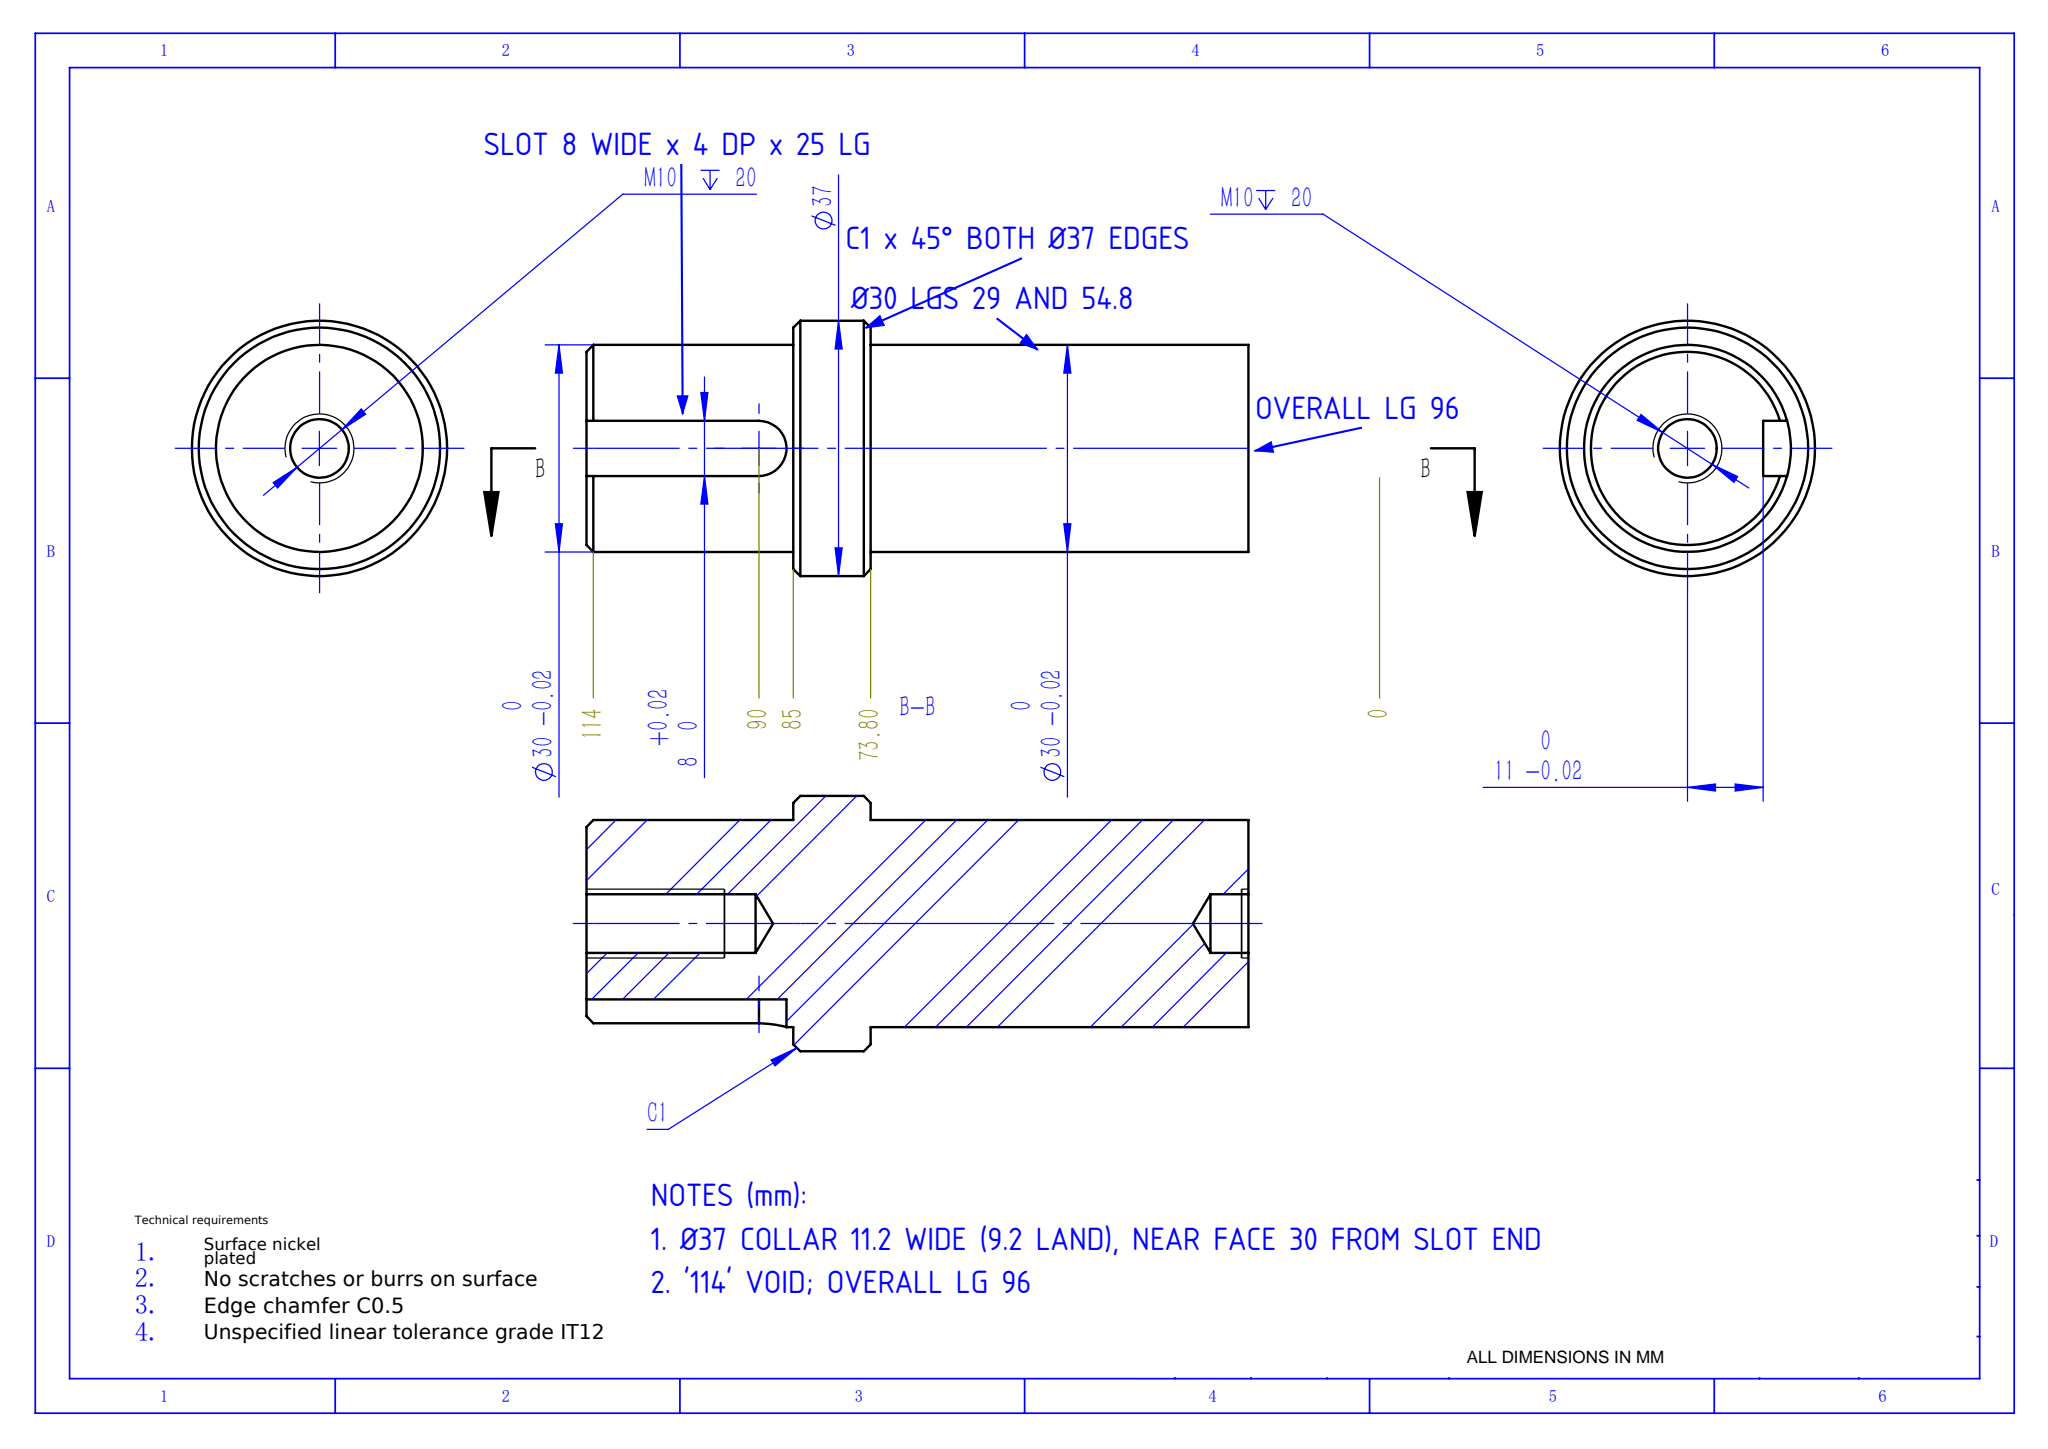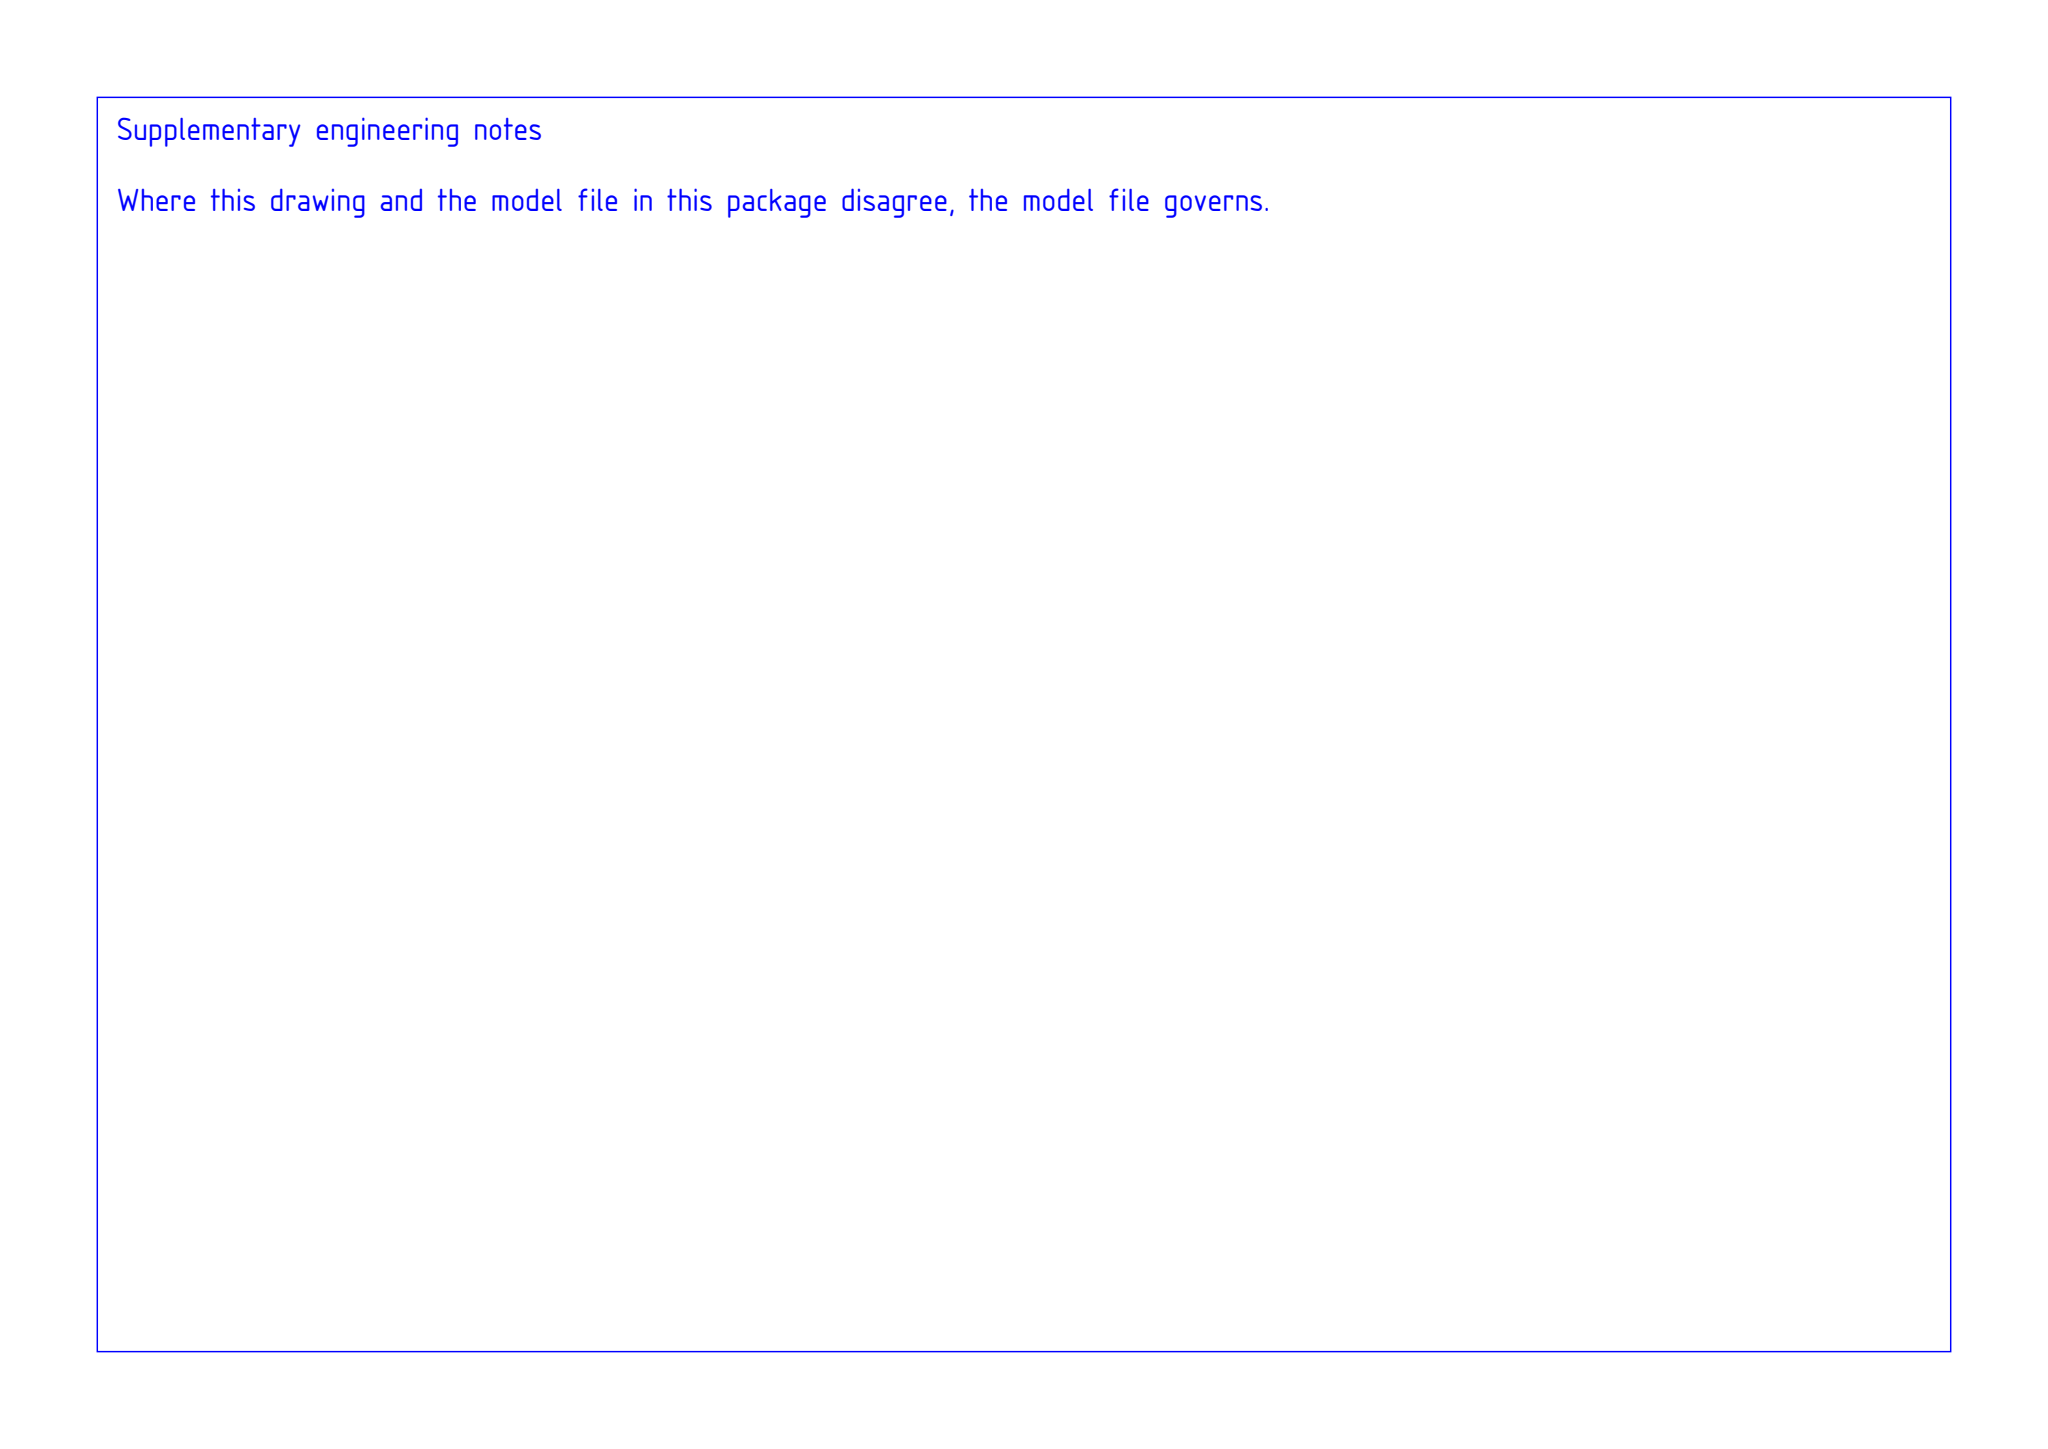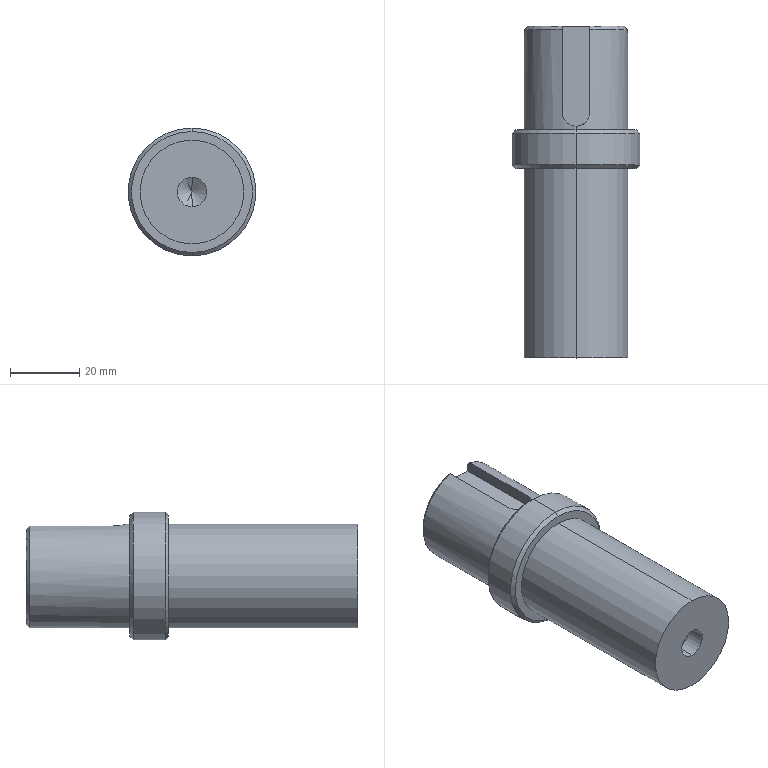Part | SolidWorks | mm | 1 solid | 28 faces | box 37 x 96 x 37 mm | volume 69168 mm3 | cylinder 11 | cone 10 | plane 7 | commonest cylinder face diameters 8.5 x4 30 x4 37 x2 8 x1
Drawing notes:
OVERALL LG 96 FROM LH END FACE; RH Ø30 SECTION 25.2 LG PAST FLANGE | from the solid: bbox_xyz y=96 overall; flange y=54.8..66.0 (Ø37 9.2 lg), Ø30 cyl y=66.0..96.0 => 30.0? RH face plane y=96.0, flange RH face y=66.0
Ø37 COLLAR 11.2 WIDE (9.2 LAND), NEAR FACE 30 FROM SLOT END | from the solid: Ø37 cyl len 9.2 between y-planes 54.8 and 66.0; end face y=96; 96-66=30
SLOT 8 WIDE x 4 DP x 25 LG FROM SLOT END FACE, R4 CLOSED END | from the solid: x-planes 14.5/22.5 = 8 wide; z-plane 29.5 vs Ø30 top 33.5 = 4 dp; Ø8 z-cyl at y=71 to end y=96 = 25, R4
Ø30 LGS: 29 SLOT END TO COLLAR, 54.8 COLLAR TO OPP END | from the solid: Ø30 cylinders len 29.0 (y 66-95) and 54.8 (y 0-54.8)
BOTH Ø37 COLLAR EDGES C1 x 45° (Ø37 TO Ø35) | from the solid: 90° cones ref dia 37 and 35 at collar faces = 1 mm chamfer
'114' VOID; OVERALL LG 96 | from the solid: bbox y = 96.0 overall
build123d program:
from build123d import *

# Parameters (mm, degrees)
SKETCH11_R             = 20
ROUND_STEEL_40_1_DEPTH = 115
M10_TAPPED_HOLE1_D     = 8.5
M10_TAPPED_HOLE1_DEPTH = 24.5
M10_TAPPED_HOLE1_TIP   = 2.554
CUT_EXTRUDE11_DEPTH    = 4
CHAMFER1_SIZE          = 1
M10_TAPPED_HOLE2_D     = 8.5
M10_TAPPED_HOLE2_DEPTH = 24.5
M10_TAPPED_HOLE2_TIP   = 2.554
SKETCH14_R             = 24.282
CUT_EXTRUDE1_DEPTH     = 19


with BuildPart() as part:
    # Sketch11 → Round Steel 40_1 (new body)
    with BuildSketch(Plane(origin=(0, 0, 0), x_dir=(-1, 0, 0), z_dir=(0, 1, 0))):
        Circle(SKETCH11_R)
    extrude(amount=ROUND_STEEL_40_1_DEPTH)

    # Sketch3 → Cut-Revolve1 (revolve, cut)
    with BuildSketch(Plane.XY, mode=Mode.PRIVATE) as cut_revolve1_sk:
        Polygon((-15, 73.8), (-18.5, 73.8), (-18.5, 85), (-15, 85), (-15, 115), (-20, 115), (-20, 0), (-15, 0), align=None)
    revolve(cut_revolve1_sk.sketch.rotate(Axis((0, 0, 0), (0, 1, 0)), 270), axis=Axis((0, 0, 0), (0, 1, 0)), mode=Mode.SUBTRACT)

    # M10 Tapped Hole1
    with Locations(Plane(origin=(0, 0, 0), x_dir=(-1, 0, 0), z_dir=(0, -1, 0))):
        with Locations((0, 0)):
            Hole(M10_TAPPED_HOLE1_D / 2, depth=M10_TAPPED_HOLE1_DEPTH)
            with Locations((0, 0, -(M10_TAPPED_HOLE1_DEPTH + M10_TAPPED_HOLE1_TIP / 2))):  # 118° drill point
                Cone(0, M10_TAPPED_HOLE1_D / 2, M10_TAPPED_HOLE1_TIP, mode=Mode.SUBTRACT)

    # Sketch31 → Cut-Extrude11 (cut)
    with BuildSketch(Plane(origin=(-0.7499, 115, 15), x_dir=(0, 1, 0), z_dir=(0, 0, -1))):
        with BuildLine():
            Line((0, 4.75), (-25, 4.75))
            ThreePointArc((-25, 4.75), (-29, 0.7499), (-25, -3.25))
            Line((-25, -3.25), (0, -3.25))
            ThreePointArc((0, -3.25), (4, 0.7499), (0, 4.75))
        make_face()
    extrude(amount=CUT_EXTRUDE11_DEPTH, mode=Mode.SUBTRACT)

    # Chamfer1
    chamfer1_edges = [part.edges().sort_by_distance(p)[0] for p in [
        (14.864, 115, -2.018),
        (0, 0, 15),
        (0, 73.8, 18.5),
        (0, 85, 18.5),
    ]]
    chamfer(chamfer1_edges, length=CHAMFER1_SIZE)

    # M10 Tapped Hole2
    with Locations(Plane(origin=(0, 115, 0), x_dir=(1, 0, 0), z_dir=(0, 1, 0))):
        with Locations((0, 0)):
            Hole(M10_TAPPED_HOLE2_D / 2, depth=M10_TAPPED_HOLE2_DEPTH)
            with Locations((0, 0, -(M10_TAPPED_HOLE2_DEPTH + M10_TAPPED_HOLE2_TIP / 2))):  # 118° drill point
                Cone(0, M10_TAPPED_HOLE2_D / 2, M10_TAPPED_HOLE2_TIP, mode=Mode.SUBTRACT)

    # Sketch14 → Cut-Extrude1 (cut)
    with BuildSketch(Plane(origin=(0, 0, 0), x_dir=(-1, 0, 0), z_dir=(0, -1, 0))):
        Circle(SKETCH14_R)
    extrude(amount=-CUT_EXTRUDE1_DEPTH, mode=Mode.SUBTRACT)


solid = part.part
STEP:
#1=CARTESIAN_POINT('',(0.,24.5,4.25));
#2=VERTEX_POINT('',#1);
#3=CARTESIAN_POINT('',(0.,24.5,-4.25));
#4=VERTEX_POINT('',#3);
#5=CARTESIAN_POINT('',(0.,24.5,0.));
#6=DIRECTION('',(0.,-1.,0.));
#7=DIRECTION('',(0.,0.,-1.));
#8=AXIS2_PLACEMENT_3D('',#5,#6,#7);
#9=CIRCLE('',#8,4.25);
#10=EDGE_CURVE('',#2,#4,#9,.T.);
#11=ORIENTED_EDGE('',*,*,#10,.F.);
#12=CARTESIAN_POINT('',(0.,19.,4.25));
#13=VERTEX_POINT('',#12);
#14=CARTESIAN_POINT('',(0.,0.,4.25));
#15=DIRECTION('',(0.,-1.,0.));
#16=VECTOR('',#15,1000.);
#17=LINE('',#14,#16);
#18=EDGE_CURVE('',#2,#13,#17,.T.);
#19=ORIENTED_EDGE('',*,*,#18,.T.);
#20=CARTESIAN_POINT('',(0.,19.,-4.25));
#21=VERTEX_POINT('',#20);
#22=CARTESIAN_POINT('',(0.,19.,0.));
#23=DIRECTION('',(0.,1.,0.));
#24=DIRECTION('',(0.,0.,-1.));
#25=AXIS2_PLACEMENT_3D('',#22,#23,#24);
#26=CIRCLE('',#25,4.25);
#27=EDGE_CURVE('',#21,#13,#26,.T.);
#28=ORIENTED_EDGE('',*,*,#27,.F.);
#29=CARTESIAN_POINT('',(0.,0.,-4.25));
#30=DIRECTION('',(0.,-1.,0.));
#31=VECTOR('',#30,1000.);
#32=LINE('',#29,#31);
#33=EDGE_CURVE('',#4,#21,#32,.T.);
#34=ORIENTED_EDGE('',*,*,#33,.F.);
#35=EDGE_LOOP('',(#11,#19,#28,#34));
#36=FACE_OUTER_BOUND('',#35,.T.);
#37=CARTESIAN_POINT('',(0.,0.,0.));
#38=DIRECTION('',(0.,-1.,0.));
#39=DIRECTION('',(0.,0.,-1.));
#40=AXIS2_PLACEMENT_3D('',#37,#38,#39);
#41=CYLINDRICAL_SURFACE('',#40,4.25);
#42=ADVANCED_FACE('',(#36),#41,.F.);
#43=CARTESIAN_POINT('',(-0.,27.054,0.));
#44=VERTEX_POINT('',#43);
#45=CARTESIAN_POINT('',(0.,24.5,-4.25));
#46=DIRECTION('',(0.,-0.515,-0.8572));
#47=VECTOR('',#46,1000.);
#48=LINE('',#45,#47);
#49=EDGE_CURVE('',#44,#4,#48,.T.);
#50=ORIENTED_EDGE('',*,*,#49,.F.);
#51=CARTESIAN_POINT('',(0.,24.5,4.25));
#52=DIRECTION('',(0.,-0.515,0.8572));
#53=VECTOR('',#52,1000.);
#54=LINE('',#51,#53);
#55=EDGE_CURVE('',#44,#2,#54,.T.);
#56=ORIENTED_EDGE('',*,*,#55,.T.);
#57=ORIENTED_EDGE('',*,*,#10,.T.);
#58=EDGE_LOOP('',(#50,#56,#57));
#59=FACE_OUTER_BOUND('',#58,.T.);
#60=CARTESIAN_POINT('',(0.,24.5,0.));
#61=DIRECTION('',(0.,-1.,0.));
#62=DIRECTION('',(0.,0.,-1.));
#63=AXIS2_PLACEMENT_3D('',#60,#61,#62);
#64=CONICAL_SURFACE('',#63,4.25,1.03);
#65=ADVANCED_FACE('',(#59),#64,.F.);
#66=CARTESIAN_POINT('',(0.,90.5,-4.25));
#67=VERTEX_POINT('',#66);
#68=CARTESIAN_POINT('',(0.,90.5,4.25));
#69=VERTEX_POINT('',#68);
#70=CARTESIAN_POINT('',(0.,90.5,0.));
#71=DIRECTION('',(0.,1.,0.));
#72=DIRECTION('',(0.,0.,1.));
#73=AXIS2_PLACEMENT_3D('',#70,#71,#72);
#74=CIRCLE('',#73,4.25);
#75=EDGE_CURVE('',#67,#69,#74,.T.);
#76=ORIENTED_EDGE('',*,*,#75,.F.);
#77=CARTESIAN_POINT('',(0.,115.,-4.25));
#78=VERTEX_POINT('',#77);
#79=CARTESIAN_POINT('',(0.,115.,-4.25));
#80=DIRECTION('',(0.,1.,0.));
#81=VECTOR('',#80,1000.);
#82=LINE('',#79,#81);
#83=EDGE_CURVE('',#67,#78,#82,.T.);
#84=ORIENTED_EDGE('',*,*,#83,.T.);
#85=CARTESIAN_POINT('',(0.,115.,4.25));
#86=VERTEX_POINT('',#85);
#87=CARTESIAN_POINT('',(0.,115.,0.));
#88=DIRECTION('',(0.,1.,0.));
#89=DIRECTION('',(0.,0.,1.));
#90=AXIS2_PLACEMENT_3D('',#87,#88,#89);
#91=CIRCLE('',#90,4.25);
#92=EDGE_CURVE('',#78,#86,#91,.T.);
#93=ORIENTED_EDGE('',*,*,#92,.T.);
#94=CARTESIAN_POINT('',(0.,115.,4.25));
#95=DIRECTION('',(0.,1.,0.));
#96=VECTOR('',#95,1000.);
#97=LINE('',#94,#96);
#98=EDGE_CURVE('',#69,#86,#97,.T.);
#99=ORIENTED_EDGE('',*,*,#98,.F.);
#100=EDGE_LOOP('',(#76,#84,#93,#99));
#101=FACE_OUTER_BOUND('',#100,.T.);
#102=CARTESIAN_POINT('',(0.,115.,0.));
#103=DIRECTION('',(0.,1.,0.));
#104=DIRECTION('',(0.,0.,1.));
#105=AXIS2_PLACEMENT_3D('',#102,#103,#104);
#106=CYLINDRICAL_SURFACE('',#105,4.25);
#107=ADVANCED_FACE('',(#101),#106,.F.);
#108=CARTESIAN_POINT('',(-0.,87.946,0.));
#109=VERTEX_POINT('',#108);
#110=CARTESIAN_POINT('',(0.,90.5,4.25));
#111=DIRECTION('',(0.,0.515,0.8572));
#112=VECTOR('',#111,1000.);
#113=LINE('',#110,#112);
#114=EDGE_CURVE('',#109,#69,#113,.T.);
#115=ORIENTED_EDGE('',*,*,#114,.F.);
#116=CARTESIAN_POINT('',(0.,90.5,-4.25));
#117=DIRECTION('',(0.,0.515,-0.8572));
#118=VECTOR('',#117,1000.);
#119=LINE('',#116,#118);
#120=EDGE_CURVE('',#109,#67,#119,.T.);
#121=ORIENTED_EDGE('',*,*,#120,.T.);
#122=ORIENTED_EDGE('',*,*,#75,.T.);
#123=EDGE_LOOP('',(#115,#121,#122));
#124=FACE_OUTER_BOUND('',#123,.T.);
#125=CARTESIAN_POINT('',(0.,90.5,0.));
#126=DIRECTION('',(0.,1.,0.));
#127=DIRECTION('',(0.,0.,1.));
#128=AXIS2_PLACEMENT_3D('',#125,#126,#127);
#129=CONICAL_SURFACE('',#128,4.25,1.03);
#130=ADVANCED_FACE('',(#124),#129,.F.);
#131=CARTESIAN_POINT('',(0.,115.,-14.));
#132=VERTEX_POINT('',#131);
#133=CARTESIAN_POINT('',(-4.,115.,13.416));
#134=VERTEX_POINT('',#133);
#135=CARTESIAN_POINT('',(0.,115.,0.));
#136=DIRECTION('',(0.,1.,0.));
#137=DIRECTION('',(0.,0.,1.));
#138=AXIS2_PLACEMENT_3D('',#135,#136,#137);
#139=CIRCLE('',#138,14.);
#140=EDGE_CURVE('',#132,#134,#139,.T.);
#141=ORIENTED_EDGE('',*,*,#140,.F.);
#142=CARTESIAN_POINT('',(0.,114.,-15.));
#143=VERTEX_POINT('',#142);
#144=CARTESIAN_POINT('',(0.,114.,-15.));
#145=DIRECTION('',(0.,-0.7071,-0.7071));
#146=VECTOR('',#145,1000.);
#147=LINE('',#144,#146);
#148=EDGE_CURVE('',#132,#143,#147,.T.);
#149=ORIENTED_EDGE('',*,*,#148,.T.);
#150=CARTESIAN_POINT('',(-4.,114.,14.457));
#151=VERTEX_POINT('',#150);
#152=CARTESIAN_POINT('',(0.,114.,0.));
#153=DIRECTION('',(0.,-1.,0.));
#154=DIRECTION('',(0.,0.,1.));
#155=AXIS2_PLACEMENT_3D('',#152,#153,#154);
#156=CIRCLE('',#155,15.);
#157=EDGE_CURVE('',#151,#143,#156,.T.);
#158=ORIENTED_EDGE('',*,*,#157,.F.);
#159=CARTESIAN_POINT('',(-4.,115.,13.416));
#160=CARTESIAN_POINT('',(-4.,114.667,13.764));
#161=CARTESIAN_POINT('',(-4.,114.334,14.11));
#162=CARTESIAN_POINT('',(-4.,114.,14.457));
#163=B_SPLINE_CURVE_WITH_KNOTS('',3,(#159,#160,#161,#162),.UNSPECIFIED.,.F.,.F.,(4,4),(0.,0.001443),.UNSPECIFIED.);
#164=EDGE_CURVE('',#134,#151,#163,.T.);
#165=ORIENTED_EDGE('',*,*,#164,.F.);
#166=EDGE_LOOP('',(#141,#149,#158,#165));
#167=FACE_OUTER_BOUND('',#166,.T.);
#168=CARTESIAN_POINT('',(0.,114.,0.));
#169=DIRECTION('',(0.,-1.,0.));
#170=DIRECTION('',(0.,0.,-1.));
#171=AXIS2_PLACEMENT_3D('',#168,#169,#170);
#172=CONICAL_SURFACE('',#171,15.,0.7854);
#173=ADVANCED_FACE('',(#167),#172,.T.);
#174=CARTESIAN_POINT('',(0.,85.,17.5));
#175=VERTEX_POINT('',#174);
#176=CARTESIAN_POINT('',(0.,85.,-17.5));
#177=VERTEX_POINT('',#176);
#178=CARTESIAN_POINT('',(0.,85.,0.));
#179=DIRECTION('',(0.,1.,0.));
#180=DIRECTION('',(0.,0.,1.));
#181=AXIS2_PLACEMENT_3D('',#178,#179,#180);
#182=CIRCLE('',#181,17.5);
#183=EDGE_CURVE('',#175,#177,#182,.T.);
#184=ORIENTED_EDGE('',*,*,#183,.F.);
#185=CARTESIAN_POINT('',(0.,84.,18.5));
#186=VERTEX_POINT('',#185);
#187=CARTESIAN_POINT('',(0.,84.,18.5));
#188=DIRECTION('',(0.,-0.7071,0.7071));
#189=VECTOR('',#188,1000.);
#190=LINE('',#187,#189);
#191=EDGE_CURVE('',#175,#186,#190,.T.);
#192=ORIENTED_EDGE('',*,*,#191,.T.);
#193=CARTESIAN_POINT('',(0.,84.,-18.5));
#194=VERTEX_POINT('',#193);
#195=CARTESIAN_POINT('',(0.,84.,0.));
#196=DIRECTION('',(0.,-1.,0.));
#197=DIRECTION('',(0.,0.,1.));
#198=AXIS2_PLACEMENT_3D('',#195,#196,#197);
#199=CIRCLE('',#198,18.5);
#200=EDGE_CURVE('',#194,#186,#199,.T.);
#201=ORIENTED_EDGE('',*,*,#200,.F.);
#202=CARTESIAN_POINT('',(0.,84.,-18.5));
#203=DIRECTION('',(0.,-0.7071,-0.7071));
#204=VECTOR('',#203,1000.);
#205=LINE('',#202,#204);
#206=EDGE_CURVE('',#177,#194,#205,.T.);
#207=ORIENTED_EDGE('',*,*,#206,.F.);
#208=EDGE_LOOP('',(#184,#192,#201,#207));
#209=FACE_OUTER_BOUND('',#208,.T.);
#210=CARTESIAN_POINT('',(0.,84.,0.));
#211=DIRECTION('',(0.,-1.,0.));
#212=DIRECTION('',(0.,0.,-1.));
#213=AXIS2_PLACEMENT_3D('',#210,#211,#212);
#214=CONICAL_SURFACE('',#213,18.5,0.7854);
#215=ADVANCED_FACE('',(#209),#214,.T.);
#216=CARTESIAN_POINT('',(0.,73.8,-17.5));
#217=VERTEX_POINT('',#216);
#218=CARTESIAN_POINT('',(0.,73.8,17.5));
#219=VERTEX_POINT('',#218);
#220=CARTESIAN_POINT('',(0.,73.8,0.));
#221=DIRECTION('',(0.,-1.,0.));
#222=DIRECTION('',(0.,0.,-1.));
#223=AXIS2_PLACEMENT_3D('',#220,#221,#222);
#224=CIRCLE('',#223,17.5);
#225=EDGE_CURVE('',#217,#219,#224,.T.);
#226=ORIENTED_EDGE('',*,*,#225,.F.);
#227=CARTESIAN_POINT('',(0.,74.8,-18.5));
#228=VERTEX_POINT('',#227);
#229=CARTESIAN_POINT('',(0.,73.8,-17.5));
#230=DIRECTION('',(0.,0.7071,-0.7071));
#231=VECTOR('',#230,1000.);
#232=LINE('',#229,#231);
#233=EDGE_CURVE('',#217,#228,#232,.T.);
#234=ORIENTED_EDGE('',*,*,#233,.T.);
#235=CARTESIAN_POINT('',(0.,74.8,18.5));
#236=VERTEX_POINT('',#235);
#237=CARTESIAN_POINT('',(0.,74.8,0.));
#238=DIRECTION('',(0.,1.,0.));
#239=DIRECTION('',(0.,0.,-1.));
#240=AXIS2_PLACEMENT_3D('',#237,#238,#239);
#241=CIRCLE('',#240,18.5);
#242=EDGE_CURVE('',#236,#228,#241,.T.);
#243=ORIENTED_EDGE('',*,*,#242,.F.);
#244=CARTESIAN_POINT('',(0.,73.8,17.5));
#245=DIRECTION('',(0.,0.7071,0.7071));
#246=VECTOR('',#245,1000.);
#247=LINE('',#244,#246);
#248=EDGE_CURVE('',#219,#236,#247,.T.);
#249=ORIENTED_EDGE('',*,*,#248,.F.);
#250=EDGE_LOOP('',(#226,#234,#243,#249));
#251=FACE_OUTER_BOUND('',#250,.T.);
#252=CARTESIAN_POINT('',(0.,73.8,0.));
#253=DIRECTION('',(0.,1.,0.));
#254=DIRECTION('',(0.,0.,1.));
#255=AXIS2_PLACEMENT_3D('',#252,#253,#254);
#256=CONICAL_SURFACE('',#255,17.5,0.7854);
#257=ADVANCED_FACE('',(#251),#256,.T.);
#258=ORIENTED_EDGE('',*,*,#200,.T.);
#259=CARTESIAN_POINT('',(0.,0.,18.5));
#260=DIRECTION('',(0.,-1.,0.));
#261=VECTOR('',#260,1000.);
#262=LINE('',#259,#261);
#263=EDGE_CURVE('',#186,#236,#262,.T.);
#264=ORIENTED_EDGE('',*,*,#263,.T.);
#265=ORIENTED_EDGE('',*,*,#242,.T.);
#266=CARTESIAN_POINT('',(0.,0.,-18.5));
#267=DIRECTION('',(0.,-1.,0.));
#268=VECTOR('',#267,1000.);
#269=LINE('',#266,#268);
#270=EDGE_CURVE('',#194,#228,#269,.T.);
#271=ORIENTED_EDGE('',*,*,#270,.F.);
#272=EDGE_LOOP('',(#258,#264,#265,#271));
#273=FACE_OUTER_BOUND('',#272,.T.);
#274=CARTESIAN_POINT('',(0.,0.,0.));
#275=DIRECTION('',(0.,-1.,0.));
#276=DIRECTION('',(0.,0.,-1.));
#277=AXIS2_PLACEMENT_3D('',#274,#275,#276);
#278=CYLINDRICAL_SURFACE('',#277,18.5);
#279=ADVANCED_FACE('',(#273),#278,.T.);
#280=CARTESIAN_POINT('',(4.,90.,14.457));
#281=VERTEX_POINT('',#280);
#282=CARTESIAN_POINT('',(0.,86.,15.));
#283=VERTEX_POINT('',#282);
#284=CARTESIAN_POINT('',(4.,90.,14.457));
#285=CARTESIAN_POINT('',(4.,89.734,14.457));
#286=CARTESIAN_POINT('',(3.974,89.473,14.464));
#287=CARTESIAN_POINT('',(3.871,88.96,14.492));
#288=CARTESIAN_POINT('',(3.794,88.706,14.513));
#289=CARTESIAN_POINT('',(3.593,88.222,14.564));
#290=CARTESIAN_POINT('',(3.47,87.992,14.594));
#291=CARTESIAN_POINT('',(3.179,87.558,14.66));
#292=CARTESIAN_POINT('',(3.011,87.354,14.696));
#293=CARTESIAN_POINT('',(2.644,86.987,14.766));
#294=CARTESIAN_POINT('',(2.443,86.822,14.801));
#295=CARTESIAN_POINT('',(2.006,86.529,14.867));
#296=CARTESIAN_POINT('',(1.775,86.406,14.897));
#297=CARTESIAN_POINT('',(1.293,86.206,14.946));
#298=CARTESIAN_POINT('',(1.04,86.129,14.966));
#299=CARTESIAN_POINT('',(0.5228,86.026,14.993));
#300=CARTESIAN_POINT('',(0.2623,86.,15.));
#301=CARTESIAN_POINT('',(0.,86.,15.));
#302=B_SPLINE_CURVE_WITH_KNOTS('',3,(#284,#285,#286,#287,#288,#289,#290,#291,#292,#293,#294,#295,#296,#297,#298,#299,#300,#301),.UNSPECIFIED.,.F.,.F.,(4,2,2,2,2,2,2,2,4),(0.,0.0007854,0.001571,0.002356,0.003142,0.003927,0.004712,0.005498,0.006283),.UNSPECIFIED.);
#303=EDGE_CURVE('',#281,#283,#302,.T.);
#304=ORIENTED_EDGE('',*,*,#303,.T.);
#305=CARTESIAN_POINT('',(0.,85.,15.));
#306=VERTEX_POINT('',#305);
#307=CARTESIAN_POINT('',(0.,0.,15.));
#308=DIRECTION('',(0.,-1.,0.));
#309=VECTOR('',#308,1000.);
#310=LINE('',#307,#309);
#311=EDGE_CURVE('',#283,#306,#310,.T.);
#312=ORIENTED_EDGE('',*,*,#311,.T.);
#313=CARTESIAN_POINT('',(0.,85.,-15.));
#314=VERTEX_POINT('',#313);
#315=CARTESIAN_POINT('',(0.,85.,0.));
#316=DIRECTION('',(0.,-1.,0.));
#317=DIRECTION('',(0.,0.,-1.));
#318=AXIS2_PLACEMENT_3D('',#315,#316,#317);
#319=CIRCLE('',#318,15.);
#320=EDGE_CURVE('',#314,#306,#319,.T.);
#321=ORIENTED_EDGE('',*,*,#320,.F.);
#322=CARTESIAN_POINT('',(0.,0.,-15.));
#323=DIRECTION('',(0.,-1.,0.));
#324=VECTOR('',#323,1000.);
#325=LINE('',#322,#324);
#326=EDGE_CURVE('',#143,#314,#325,.T.);
#327=ORIENTED_EDGE('',*,*,#326,.F.);
#328=CARTESIAN_POINT('',(4.,114.,14.457));
#329=VERTEX_POINT('',#328);
#330=CARTESIAN_POINT('',(0.,114.,0.));
#331=DIRECTION('',(0.,-1.,0.));
#332=DIRECTION('',(0.,0.,1.));
#333=AXIS2_PLACEMENT_3D('',#330,#331,#332);
#334=CIRCLE('',#333,15.);
#335=EDGE_CURVE('',#143,#329,#334,.T.);
#336=ORIENTED_EDGE('',*,*,#335,.T.);
#337=CARTESIAN_POINT('',(4.,-0.,14.457));
#338=DIRECTION('',(0.,-1.,0.));
#339=VECTOR('',#338,1000.);
#340=LINE('',#337,#339);
#341=EDGE_CURVE('',#329,#281,#340,.T.);
#342=ORIENTED_EDGE('',*,*,#341,.T.);
#343=EDGE_LOOP('',(#304,#312,#321,#327,#336,#342));
#344=FACE_OUTER_BOUND('',#343,.T.);
#345=CARTESIAN_POINT('',(0.,0.,0.));
#346=DIRECTION('',(0.,-1.,0.));
#347=DIRECTION('',(0.,0.,-1.));
#348=AXIS2_PLACEMENT_3D('',#345,#346,#347);
#349=CYLINDRICAL_SURFACE('',#348,15.);
#350=ADVANCED_FACE('',(#344),#349,.T.);
#351=CARTESIAN_POINT('',(0.,73.8,-15.));
#352=VERTEX_POINT('',#351);
#353=CARTESIAN_POINT('',(0.,73.8,15.));
#354=VERTEX_POINT('',#353);
#355=CARTESIAN_POINT('',(0.,73.8,0.));
#356=DIRECTION('',(0.,-1.,0.));
#357=DIRECTION('',(0.,0.,-1.));
#358=AXIS2_PLACEMENT_3D('',#355,#356,#357);
#359=CIRCLE('',#358,15.);
#360=EDGE_CURVE('',#352,#354,#359,.T.);
#361=ORIENTED_EDGE('',*,*,#360,.T.);
#362=CARTESIAN_POINT('',(0.,19.,15.));
#363=VERTEX_POINT('',#362);
#364=CARTESIAN_POINT('',(0.,0.,15.));
#365=DIRECTION('',(0.,-1.,0.));
#366=VECTOR('',#365,1000.);
#367=LINE('',#364,#366);
#368=EDGE_CURVE('',#354,#363,#367,.T.);
#369=ORIENTED_EDGE('',*,*,#368,.T.);
#370=CARTESIAN_POINT('',(0.,19.,-15.));
#371=VERTEX_POINT('',#370);
#372=CARTESIAN_POINT('',(0.,19.,0.));
#373=DIRECTION('',(0.,1.,0.));
#374=DIRECTION('',(0.,0.,-1.));
#375=AXIS2_PLACEMENT_3D('',#372,#373,#374);
#376=CIRCLE('',#375,15.);
#377=EDGE_CURVE('',#363,#371,#376,.T.);
#378=ORIENTED_EDGE('',*,*,#377,.T.);
#379=CARTESIAN_POINT('',(0.,0.,-15.));
#380=DIRECTION('',(0.,-1.,0.));
#381=VECTOR('',#380,1000.);
#382=LINE('',#379,#381);
#383=EDGE_CURVE('',#352,#371,#382,.T.);
#384=ORIENTED_EDGE('',*,*,#383,.F.);
#385=EDGE_LOOP('',(#361,#369,#378,#384));
#386=FACE_OUTER_BOUND('',#385,.T.);
#387=CARTESIAN_POINT('',(0.,0.,0.));
#388=DIRECTION('',(0.,-1.,0.));
#389=DIRECTION('',(0.,0.,-1.));
#390=AXIS2_PLACEMENT_3D('',#387,#388,#389);
#391=CYLINDRICAL_SURFACE('',#390,15.);
#392=ADVANCED_FACE('',(#386),#391,.T.);
#393=ORIENTED_EDGE('',*,*,#368,.F.);
#394=CARTESIAN_POINT('',(0.,73.8,0.));
#395=DIRECTION('',(0.,-1.,0.));
#396=DIRECTION('',(0.,0.,-1.));
#397=AXIS2_PLACEMENT_3D('',#394,#395,#396);
#398=CIRCLE('',#397,15.);
#399=EDGE_CURVE('',#354,#352,#398,.T.);
#400=ORIENTED_EDGE('',*,*,#399,.T.);
#401=ORIENTED_EDGE('',*,*,#383,.T.);
#402=CARTESIAN_POINT('',(0.,19.,0.));
#403=DIRECTION('',(0.,1.,0.));
#404=DIRECTION('',(0.,0.,-1.));
#405=AXIS2_PLACEMENT_3D('',#402,#403,#404);
#406=CIRCLE('',#405,15.);
#407=EDGE_CURVE('',#371,#363,#406,.T.);
#408=ORIENTED_EDGE('',*,*,#407,.T.);
#409=EDGE_LOOP('',(#393,#400,#401,#408));
#410=FACE_OUTER_BOUND('',#409,.T.);
#411=CARTESIAN_POINT('',(0.,0.,0.));
#412=DIRECTION('',(0.,-1.,0.));
#413=DIRECTION('',(0.,0.,-1.));
#414=AXIS2_PLACEMENT_3D('',#411,#412,#413);
#415=CYLINDRICAL_SURFACE('',#414,15.);
#416=ADVANCED_FACE('',(#410),#415,.T.);
#417=ORIENTED_EDGE('',*,*,#311,.F.);
#418=CARTESIAN_POINT('',(-4.,90.,14.457));
#419=VERTEX_POINT('',#418);
#420=CARTESIAN_POINT('',(0.,86.,15.));
#421=CARTESIAN_POINT('',(-0.262,86.,15.));
#422=CARTESIAN_POINT('',(-0.5282,86.026,14.993));
#423=CARTESIAN_POINT('',(-1.042,86.129,14.966));
#424=CARTESIAN_POINT('',(-1.292,86.205,14.946));
#425=CARTESIAN_POINT('',(-2.02,86.508,14.871));
#426=CARTESIAN_POINT('',(-2.459,86.802,14.802));
#427=CARTESIAN_POINT('',(-3.014,87.357,14.695));
#428=CARTESIAN_POINT('',(-3.178,87.557,14.66));
#429=CARTESIAN_POINT('',(-3.467,87.989,14.594));
#430=CARTESIAN_POINT('',(-3.593,88.223,14.564));
#431=CARTESIAN_POINT('',(-3.794,88.705,14.513));
#432=CARTESIAN_POINT('',(-3.87,88.954,14.492));
#433=CARTESIAN_POINT('',(-3.973,89.469,14.464));
#434=CARTESIAN_POINT('',(-4.,89.735,14.457));
#435=CARTESIAN_POINT('',(-4.,90.,14.457));
#436=B_SPLINE_CURVE_WITH_KNOTS('',3,(#420,#421,#422,#423,#424,#425,#426,#427,#428,#429,#430,#431,#432,#433,#434,#435),.UNSPECIFIED.,.F.,.F.,(4,2,2,2,2,2,2,4),(0.006283,0.007068,0.007852,0.009421,0.01021,0.01099,0.01177,0.01256),.UNSPECIFIED.);
#437=EDGE_CURVE('',#283,#419,#436,.T.);
#438=ORIENTED_EDGE('',*,*,#437,.T.);
#439=CARTESIAN_POINT('',(-4.,0.,14.457));
#440=DIRECTION('',(0.,1.,0.));
#441=VECTOR('',#440,1000.);
#442=LINE('',#439,#441);
#443=EDGE_CURVE('',#419,#151,#442,.T.);
#444=ORIENTED_EDGE('',*,*,#443,.T.);
#445=ORIENTED_EDGE('',*,*,#157,.T.);
#446=ORIENTED_EDGE('',*,*,#326,.T.);
#447=CARTESIAN_POINT('',(0.,85.,0.));
#448=DIRECTION('',(0.,-1.,0.));
#449=DIRECTION('',(0.,0.,-1.));
#450=AXIS2_PLACEMENT_3D('',#447,#448,#449);
#451=CIRCLE('',#450,15.);
#452=EDGE_CURVE('',#306,#314,#451,.T.);
#453=ORIENTED_EDGE('',*,*,#452,.F.);
#454=EDGE_LOOP('',(#417,#438,#444,#445,#446,#453));
#455=FACE_OUTER_BOUND('',#454,.T.);
#456=CARTESIAN_POINT('',(0.,0.,0.));
#457=DIRECTION('',(0.,-1.,0.));
#458=DIRECTION('',(0.,0.,-1.));
#459=AXIS2_PLACEMENT_3D('',#456,#457,#458);
#460=CYLINDRICAL_SURFACE('',#459,15.);
#461=ADVANCED_FACE('',(#455),#460,.T.);
#462=CARTESIAN_POINT('',(0.,115.,0.));
#463=DIRECTION('',(0.,1.,0.));
#464=DIRECTION('',(0.,0.,1.));
#465=AXIS2_PLACEMENT_3D('',#462,#463,#464);
#466=CIRCLE('',#465,4.25);
#467=EDGE_CURVE('',#86,#78,#466,.T.);
#468=ORIENTED_EDGE('',*,*,#467,.F.);
#469=ORIENTED_EDGE('',*,*,#92,.F.);
#470=EDGE_LOOP('',(#468,#469));
#471=FACE_BOUND('',#470,.T.);
#472=CARTESIAN_POINT('',(4.,115.,11.));
#473=VERTEX_POINT('',#472);
#474=CARTESIAN_POINT('',(4.,115.,13.416));
#475=VERTEX_POINT('',#474);
#476=CARTESIAN_POINT('',(4.,115.,11.));
#477=DIRECTION('',(0.,-0.,1.));
#478=VECTOR('',#477,1000.);
#479=LINE('',#476,#478);
#480=EDGE_CURVE('',#473,#475,#479,.T.);
#481=ORIENTED_EDGE('',*,*,#480,.T.);
#482=CARTESIAN_POINT('',(0.,115.,0.));
#483=DIRECTION('',(0.,1.,0.));
#484=DIRECTION('',(0.,0.,1.));
#485=AXIS2_PLACEMENT_3D('',#482,#483,#484);
#486=CIRCLE('',#485,14.);
#487=EDGE_CURVE('',#475,#132,#486,.T.);
#488=ORIENTED_EDGE('',*,*,#487,.T.);
#489=ORIENTED_EDGE('',*,*,#140,.T.);
#490=CARTESIAN_POINT('',(-4.,115.,11.));
#491=VERTEX_POINT('',#490);
#492=CARTESIAN_POINT('',(-4.,115.,11.));
#493=DIRECTION('',(0.,-0.,1.));
#494=VECTOR('',#493,1000.);
#495=LINE('',#492,#494);
#496=EDGE_CURVE('',#491,#134,#495,.T.);
#497=ORIENTED_EDGE('',*,*,#496,.F.);
#498=CARTESIAN_POINT('',(0.,115.,11.));
#499=DIRECTION('',(1.,0.,-0.));
#500=VECTOR('',#499,1000.);
#501=LINE('',#498,#500);
#502=EDGE_CURVE('',#491,#473,#501,.T.);
#503=ORIENTED_EDGE('',*,*,#502,.T.);
#504=EDGE_LOOP('',(#481,#488,#489,#497,#503));
#505=FACE_OUTER_BOUND('',#504,.T.);
#506=CARTESIAN_POINT('',(0.,115.,0.));
#507=DIRECTION('',(0.,1.,0.));
#508=DIRECTION('',(0.,0.,1.));
#509=AXIS2_PLACEMENT_3D('',#506,#507,#508);
#510=PLANE('',#509);
#511=ADVANCED_FACE('',(#471,#505),#510,.T.);
#512=CARTESIAN_POINT('',(0.,73.8,0.));
#513=DIRECTION('',(0.,-1.,0.));
#514=DIRECTION('',(0.,0.,-1.));
#515=AXIS2_PLACEMENT_3D('',#512,#513,#514);
#516=CIRCLE('',#515,17.5);
#517=EDGE_CURVE('',#219,#217,#516,.T.);
#518=ORIENTED_EDGE('',*,*,#517,.T.);
#519=ORIENTED_EDGE('',*,*,#225,.T.);
#520=EDGE_LOOP('',(#518,#519));
#521=FACE_OUTER_BOUND('',#520,.T.);
#522=ORIENTED_EDGE('',*,*,#360,.F.);
#523=ORIENTED_EDGE('',*,*,#399,.F.);
#524=EDGE_LOOP('',(#522,#523));
#525=FACE_BOUND('',#524,.T.);
#526=CARTESIAN_POINT('',(-15.,73.8,0.));
#527=DIRECTION('',(0.,-1.,0.));
#528=DIRECTION('',(0.,0.,-1.));
#529=AXIS2_PLACEMENT_3D('',#526,#527,#528);
#530=PLANE('',#529);
#531=ADVANCED_FACE('',(#521,#525),#530,.T.);
#532=ORIENTED_EDGE('',*,*,#263,.F.);
#533=CARTESIAN_POINT('',(0.,84.,0.));
#534=DIRECTION('',(0.,-1.,0.));
#535=DIRECTION('',(0.,0.,1.));
#536=AXIS2_PLACEMENT_3D('',#533,#534,#535);
#537=CIRCLE('',#536,18.5);
#538=EDGE_CURVE('',#186,#194,#537,.T.);
#539=ORIENTED_EDGE('',*,*,#538,.T.);
#540=ORIENTED_EDGE('',*,*,#270,.T.);
#541=CARTESIAN_POINT('',(0.,74.8,0.));
#542=DIRECTION('',(0.,1.,0.));
#543=DIRECTION('',(0.,0.,-1.));
#544=AXIS2_PLACEMENT_3D('',#541,#542,#543);
#545=CIRCLE('',#544,18.5);
#546=EDGE_CURVE('',#228,#236,#545,.T.);
#547=ORIENTED_EDGE('',*,*,#546,.T.);
#548=EDGE_LOOP('',(#532,#539,#540,#547));
#549=FACE_OUTER_BOUND('',#548,.T.);
#550=CARTESIAN_POINT('',(0.,0.,0.));
#551=DIRECTION('',(0.,-1.,0.));
#552=DIRECTION('',(0.,0.,-1.));
#553=AXIS2_PLACEMENT_3D('',#550,#551,#552);
#554=CYLINDRICAL_SURFACE('',#553,18.5);
#555=ADVANCED_FACE('',(#549),#554,.T.);
#556=CARTESIAN_POINT('',(0.,85.,0.));
#557=DIRECTION('',(0.,1.,0.));
#558=DIRECTION('',(0.,0.,1.));
#559=AXIS2_PLACEMENT_3D('',#556,#557,#558);
#560=CIRCLE('',#559,17.5);
#561=EDGE_CURVE('',#177,#175,#560,.T.);
#562=ORIENTED_EDGE('',*,*,#561,.T.);
#563=ORIENTED_EDGE('',*,*,#183,.T.);
#564=EDGE_LOOP('',(#562,#563));
#565=FACE_OUTER_BOUND('',#564,.T.);
#566=ORIENTED_EDGE('',*,*,#320,.T.);
#567=ORIENTED_EDGE('',*,*,#452,.T.);
#568=EDGE_LOOP('',(#566,#567));
#569=FACE_BOUND('',#568,.T.);
#570=CARTESIAN_POINT('',(-18.5,85.,0.));
#571=DIRECTION('',(0.,1.,0.));
#572=DIRECTION('',(0.,0.,1.));
#573=AXIS2_PLACEMENT_3D('',#570,#571,#572);
#574=PLANE('',#573);
#575=ADVANCED_FACE('',(#565,#569),#574,.T.);
#576=ORIENTED_EDGE('',*,*,#341,.F.);
#577=CARTESIAN_POINT('',(4.,114.,14.457));
#578=CARTESIAN_POINT('',(4.,114.334,14.11));
#579=CARTESIAN_POINT('',(4.,114.667,13.764));
#580=CARTESIAN_POINT('',(4.,115.,13.416));
#581=B_SPLINE_CURVE_WITH_KNOTS('',3,(#577,#578,#579,#580),.UNSPECIFIED.,.F.,.F.,(4,4),(0.,0.001443),.UNSPECIFIED.);
#582=EDGE_CURVE('',#329,#475,#581,.T.);
#583=ORIENTED_EDGE('',*,*,#582,.T.);
#584=ORIENTED_EDGE('',*,*,#480,.F.);
#585=CARTESIAN_POINT('',(4.,90.,11.));
#586=VERTEX_POINT('',#585);
#587=CARTESIAN_POINT('',(4.,115.,11.));
#588=DIRECTION('',(-0.,-1.,-0.));
#589=VECTOR('',#588,1000.);
#590=LINE('',#587,#589);
#591=EDGE_CURVE('',#473,#586,#590,.T.);
#592=ORIENTED_EDGE('',*,*,#591,.T.);
#593=CARTESIAN_POINT('',(4.,90.,11.));
#594=DIRECTION('',(0.,-0.,1.));
#595=VECTOR('',#594,1000.);
#596=LINE('',#593,#595);
#597=EDGE_CURVE('',#586,#281,#596,.T.);
#598=ORIENTED_EDGE('',*,*,#597,.T.);
#599=EDGE_LOOP('',(#576,#583,#584,#592,#598));
#600=FACE_OUTER_BOUND('',#599,.T.);
#601=CARTESIAN_POINT('',(4.,115.,11.));
#602=DIRECTION('',(-1.,0.,0.));
#603=DIRECTION('',(-0.,-1.,0.));
#604=AXIS2_PLACEMENT_3D('',#601,#602,#603);
#605=PLANE('',#604);
#606=ADVANCED_FACE('',(#600),#605,.T.);
#607=ORIENTED_EDGE('',*,*,#597,.F.);
#608=CARTESIAN_POINT('',(-4.,90.,11.));
#609=VERTEX_POINT('',#608);
#610=CARTESIAN_POINT('',(-0.,90.,11.));
#611=DIRECTION('',(-0.,0.,-1.));
#612=DIRECTION('',(-1.,0.,0.));
#613=AXIS2_PLACEMENT_3D('',#610,#611,#612);
#614=CIRCLE('',#613,4.);
#615=EDGE_CURVE('',#586,#609,#614,.T.);
#616=ORIENTED_EDGE('',*,*,#615,.T.);
#617=CARTESIAN_POINT('',(-4.,90.,11.));
#618=DIRECTION('',(0.,-0.,1.));
#619=VECTOR('',#618,1000.);
#620=LINE('',#617,#619);
#621=EDGE_CURVE('',#609,#419,#620,.T.);
#622=ORIENTED_EDGE('',*,*,#621,.T.);
#623=ORIENTED_EDGE('',*,*,#437,.F.);
#624=ORIENTED_EDGE('',*,*,#303,.F.);
#625=EDGE_LOOP('',(#607,#616,#622,#623,#624));
#626=FACE_OUTER_BOUND('',#625,.T.);
#627=CARTESIAN_POINT('',(-0.,90.,11.));
#628=DIRECTION('',(0.,-0.,1.));
#629=DIRECTION('',(1.,0.,0.));
#630=AXIS2_PLACEMENT_3D('',#627,#628,#629);
#631=CYLINDRICAL_SURFACE('',#630,4.);
#632=ADVANCED_FACE('',(#626),#631,.F.);
#633=ORIENTED_EDGE('',*,*,#496,.T.);
#634=ORIENTED_EDGE('',*,*,#164,.T.);
#635=ORIENTED_EDGE('',*,*,#443,.F.);
#636=ORIENTED_EDGE('',*,*,#621,.F.);
#637=CARTESIAN_POINT('',(-4.,115.,11.));
#638=DIRECTION('',(0.,1.,0.));
#639=VECTOR('',#638,1000.);
#640=LINE('',#637,#639);
#641=EDGE_CURVE('',#609,#491,#640,.T.);
#642=ORIENTED_EDGE('',*,*,#641,.T.);
#643=EDGE_LOOP('',(#633,#634,#635,#636,#642));
#644=FACE_OUTER_BOUND('',#643,.T.);
#645=CARTESIAN_POINT('',(-4.,115.,11.));
#646=DIRECTION('',(1.,-0.,-0.));
#647=DIRECTION('',(0.,1.,0.));
#648=AXIS2_PLACEMENT_3D('',#645,#646,#647);
#649=PLANE('',#648);
#650=ADVANCED_FACE('',(#644),#649,.T.);
#651=ORIENTED_EDGE('',*,*,#641,.F.);
#652=ORIENTED_EDGE('',*,*,#615,.F.);
#653=ORIENTED_EDGE('',*,*,#591,.F.);
#654=ORIENTED_EDGE('',*,*,#502,.F.);
#655=EDGE_LOOP('',(#651,#652,#653,#654));
#656=FACE_OUTER_BOUND('',#655,.T.);
#657=CARTESIAN_POINT('',(0.,115.,11.));
#658=DIRECTION('',(0.,-0.,1.));
#659=DIRECTION('',(1.,0.,-0.));
#660=AXIS2_PLACEMENT_3D('',#657,#658,#659);
#661=PLANE('',#660);
#662=ADVANCED_FACE('',(#656),#661,.T.);
#663=ORIENTED_EDGE('',*,*,#233,.F.);
#664=ORIENTED_EDGE('',*,*,#517,.F.);
#665=ORIENTED_EDGE('',*,*,#248,.T.);
#666=ORIENTED_EDGE('',*,*,#546,.F.);
#667=EDGE_LOOP('',(#663,#664,#665,#666));
#668=FACE_OUTER_BOUND('',#667,.T.);
#669=CARTESIAN_POINT('',(0.,73.8,0.));
#670=DIRECTION('',(0.,1.,0.));
#671=DIRECTION('',(0.,0.,1.));
#672=AXIS2_PLACEMENT_3D('',#669,#670,#671);
#673=CONICAL_SURFACE('',#672,17.5,0.7854);
#674=ADVANCED_FACE('',(#668),#673,.T.);
#675=ORIENTED_EDGE('',*,*,#191,.F.);
#676=ORIENTED_EDGE('',*,*,#561,.F.);
#677=ORIENTED_EDGE('',*,*,#206,.T.);
#678=ORIENTED_EDGE('',*,*,#538,.F.);
#679=EDGE_LOOP('',(#675,#676,#677,#678));
#680=FACE_OUTER_BOUND('',#679,.T.);
#681=CARTESIAN_POINT('',(0.,84.,0.));
#682=DIRECTION('',(0.,-1.,0.));
#683=DIRECTION('',(0.,0.,-1.));
#684=AXIS2_PLACEMENT_3D('',#681,#682,#683);
#685=CONICAL_SURFACE('',#684,18.5,0.7854);
#686=ADVANCED_FACE('',(#680),#685,.T.);
#687=ORIENTED_EDGE('',*,*,#148,.F.);
#688=ORIENTED_EDGE('',*,*,#487,.F.);
#689=ORIENTED_EDGE('',*,*,#582,.F.);
#690=ORIENTED_EDGE('',*,*,#335,.F.);
#691=EDGE_LOOP('',(#687,#688,#689,#690));
#692=FACE_OUTER_BOUND('',#691,.T.);
#693=CARTESIAN_POINT('',(0.,114.,0.));
#694=DIRECTION('',(0.,-1.,0.));
#695=DIRECTION('',(0.,0.,-1.));
#696=AXIS2_PLACEMENT_3D('',#693,#694,#695);
#697=CONICAL_SURFACE('',#696,15.,0.7854);
#698=ADVANCED_FACE('',(#692),#697,.T.);
#699=ORIENTED_EDGE('',*,*,#120,.F.);
#700=ORIENTED_EDGE('',*,*,#114,.T.);
#701=CARTESIAN_POINT('',(0.,90.5,0.));
#702=DIRECTION('',(0.,1.,0.));
#703=DIRECTION('',(0.,0.,1.));
#704=AXIS2_PLACEMENT_3D('',#701,#702,#703);
#705=CIRCLE('',#704,4.25);
#706=EDGE_CURVE('',#69,#67,#705,.T.);
#707=ORIENTED_EDGE('',*,*,#706,.T.);
#708=EDGE_LOOP('',(#699,#700,#707));
#709=FACE_OUTER_BOUND('',#708,.T.);
#710=CARTESIAN_POINT('',(0.,90.5,0.));
#711=DIRECTION('',(0.,1.,0.));
#712=DIRECTION('',(0.,0.,1.));
#713=AXIS2_PLACEMENT_3D('',#710,#711,#712);
#714=CONICAL_SURFACE('',#713,4.25,1.03);
#715=ADVANCED_FACE('',(#709),#714,.F.);
#716=ORIENTED_EDGE('',*,*,#83,.F.);
#717=ORIENTED_EDGE('',*,*,#706,.F.);
#718=ORIENTED_EDGE('',*,*,#98,.T.);
#719=ORIENTED_EDGE('',*,*,#467,.T.);
#720=EDGE_LOOP('',(#716,#717,#718,#719));
#721=FACE_OUTER_BOUND('',#720,.T.);
#722=CARTESIAN_POINT('',(0.,115.,0.));
#723=DIRECTION('',(0.,1.,0.));
#724=DIRECTION('',(0.,0.,1.));
#725=AXIS2_PLACEMENT_3D('',#722,#723,#724);
#726=CYLINDRICAL_SURFACE('',#725,4.25);
#727=ADVANCED_FACE('',(#721),#726,.F.);
#728=ORIENTED_EDGE('',*,*,#407,.F.);
#729=ORIENTED_EDGE('',*,*,#377,.F.);
#730=EDGE_LOOP('',(#728,#729));
#731=FACE_OUTER_BOUND('',#730,.T.);
#732=ORIENTED_EDGE('',*,*,#27,.T.);
#733=CARTESIAN_POINT('',(0.,19.,0.));
#734=DIRECTION('',(0.,1.,0.));
#735=DIRECTION('',(0.,0.,-1.));
#736=AXIS2_PLACEMENT_3D('',#733,#734,#735);
#737=CIRCLE('',#736,4.25);
#738=EDGE_CURVE('',#13,#21,#737,.T.);
#739=ORIENTED_EDGE('',*,*,#738,.T.);
#740=EDGE_LOOP('',(#732,#739));
#741=FACE_BOUND('',#740,.T.);
#742=CARTESIAN_POINT('',(-0.,19.,0.));
#743=DIRECTION('',(0.,-1.,0.));
#744=DIRECTION('',(0.,0.,-1.));
#745=AXIS2_PLACEMENT_3D('',#742,#743,#744);
#746=PLANE('',#745);
#747=ADVANCED_FACE('',(#731,#741),#746,.T.);
#748=ORIENTED_EDGE('',*,*,#55,.F.);
#749=ORIENTED_EDGE('',*,*,#49,.T.);
#750=CARTESIAN_POINT('',(0.,24.5,0.));
#751=DIRECTION('',(0.,-1.,0.));
#752=DIRECTION('',(0.,0.,-1.));
#753=AXIS2_PLACEMENT_3D('',#750,#751,#752);
#754=CIRCLE('',#753,4.25);
#755=EDGE_CURVE('',#4,#2,#754,.T.);
#756=ORIENTED_EDGE('',*,*,#755,.T.);
#757=EDGE_LOOP('',(#748,#749,#756));
#758=FACE_OUTER_BOUND('',#757,.T.);
#759=CARTESIAN_POINT('',(0.,24.5,0.));
#760=DIRECTION('',(0.,-1.,0.));
#761=DIRECTION('',(0.,0.,-1.));
#762=AXIS2_PLACEMENT_3D('',#759,#760,#761);
#763=CONICAL_SURFACE('',#762,4.25,1.03);
#764=ADVANCED_FACE('',(#758),#763,.F.);
#765=ORIENTED_EDGE('',*,*,#18,.F.);
#766=ORIENTED_EDGE('',*,*,#755,.F.);
#767=ORIENTED_EDGE('',*,*,#33,.T.);
#768=ORIENTED_EDGE('',*,*,#738,.F.);
#769=EDGE_LOOP('',(#765,#766,#767,#768));
#770=FACE_OUTER_BOUND('',#769,.T.);
#771=CARTESIAN_POINT('',(0.,0.,0.));
#772=DIRECTION('',(0.,-1.,0.));
#773=DIRECTION('',(0.,0.,-1.));
#774=AXIS2_PLACEMENT_3D('',#771,#772,#773);
#775=CYLINDRICAL_SURFACE('',#774,4.25);
#776=ADVANCED_FACE('',(#770),#775,.F.);
#777=CLOSED_SHELL('',(#42,#65,#107,#130,#173,#215,#257,#279,#350,#392,#416,#461,#511,#531,#555,#575,#606,#632,#650,#662,#674,#686,#698,#715,#727,#747,#764,#776));
#778=MANIFOLD_SOLID_BREP('',#777);
#779=CARTESIAN_POINT('',(0.,0.,0.));
#780=DIRECTION('',(0.,0.,1.));
#781=DIRECTION('',(1.,0.,0.));
#782=AXIS2_PLACEMENT_3D('',#779,#780,#781);
#783=(LENGTH_UNIT()NAMED_UNIT(*)SI_UNIT(.MILLI.,.METRE.));
#784=UNCERTAINTY_MEASURE_WITH_UNIT(LENGTH_MEASURE(0.00001),#783,'','');
#785=(NAMED_UNIT(*)PLANE_ANGLE_UNIT()SI_UNIT($,.RADIAN.));
#786=(NAMED_UNIT(*)SI_UNIT($,.STERADIAN.)SOLID_ANGLE_UNIT());
#787=(GEOMETRIC_REPRESENTATION_CONTEXT(3)GLOBAL_UNCERTAINTY_ASSIGNED_CONTEXT((#784))GLOBAL_UNIT_ASSIGNED_CONTEXT((#783,#785,#786))REPRESENTATION_CONTEXT('',''));
#788=ADVANCED_BREP_SHAPE_REPRESENTATION('',(#778,#782),#787);